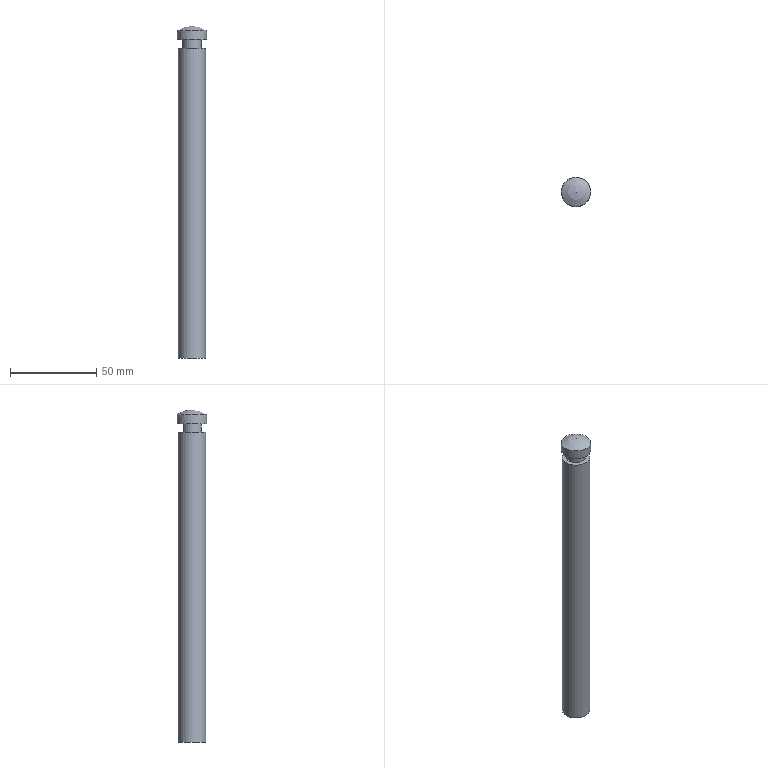Component | NX | STUD_B_2 | 1 solid | 7 faces | box 17 x 17 x 192 mm | volume 37991 mm3 | plane 3 | cylinder 3 | sphere 1 | commonest cylinder face diameters 16 x1 11 x1 17 x1
STEP:
#1=CARTESIAN_POINT('',(0.,0.,0.));
#2=DIRECTION('',(0.,0.,1.));
#3=DIRECTION('',(1.,0.,0.));
#4=AXIS2_PLACEMENT_3D('',#1,#2,#3);
#5=CARTESIAN_POINT('',(194.,-0.,10.));
#6=VERTEX_POINT('',#5);
#7=CARTESIAN_POINT('',(186.,-0.,10.));
#8=DIRECTION('',(0.,0.,1.));
#9=DIRECTION('',(1.,0.,0.));
#10=AXIS2_PLACEMENT_3D('',#7,#8,#9);
#11=CIRCLE('',#10,8.);
#12=CARTESIAN_POINT('',(186.,-0.,10.));
#13=DIRECTION('',(0.,0.,1.));
#14=DIRECTION('',(1.,0.,0.));
#15=AXIS2_PLACEMENT_3D('',#12,#13,#14);
#16=PLANE('',#15);
#17=CARTESIAN_POINT('',(0.,0.));
#18=DIRECTION('',(1.,0.));
#19=AXIS2_PLACEMENT_2D('',#17,#18);
#20=CIRCLE('',#19,8.);
#21=(GEOMETRIC_REPRESENTATION_CONTEXT(2)PARAMETRIC_REPRESENTATION_CONTEXT()REPRESENTATION_CONTEXT('',''));
#22=DEFINITIONAL_REPRESENTATION('',(#20),#21);
#23=PCURVE('',#16,#22);
#24=CARTESIAN_POINT('',(186.,-0.,202.));
#25=DIRECTION('',(0.,0.,1.));
#26=DIRECTION('',(1.,0.,0.));
#27=AXIS2_PLACEMENT_3D('',#24,#25,#26);
#28=CYLINDRICAL_SURFACE('',#27,8.);
#29=CARTESIAN_POINT('',(0.,-192.));
#30=DIRECTION('',(1.,0.));
#31=VECTOR('',#30,1.);
#32=LINE('',#29,#31);
#33=(GEOMETRIC_REPRESENTATION_CONTEXT(2)PARAMETRIC_REPRESENTATION_CONTEXT()REPRESENTATION_CONTEXT('',''));
#34=DEFINITIONAL_REPRESENTATION('',(#32),#33);
#35=PCURVE('',#28,#34);
#36=SURFACE_CURVE('',#11,(#23,#35),.PCURVE_S1.);
#37=EDGE_CURVE('',#6,#6,#36,.T.);
#38=ORIENTED_EDGE('',*,*,#37,.F.);
#39=EDGE_LOOP('',(#38));
#40=FACE_BOUND('',#39,.T.);
#41=ADVANCED_FACE('',(#40),#16,.F.);
#42=ORIENTED_EDGE('',*,*,#37,.T.);
#43=CARTESIAN_POINT('',(194.,-0.,189.));
#44=VERTEX_POINT('',#43);
#45=CARTESIAN_POINT('',(194.,-0.,10.));
#46=CARTESIAN_POINT('',(194.,-0.,189.));
#47=B_SPLINE_CURVE_WITH_KNOTS('',1,(#45,#46),.UNSPECIFIED.,.F.,.F.,(2,2),(-192.,-13.),.PIECEWISE_BEZIER_KNOTS.);
#48=CARTESIAN_POINT('',(6.283,0.));
#49=DIRECTION('',(0.,1.));
#50=VECTOR('',#49,1.);
#51=LINE('',#48,#50);
#52=(GEOMETRIC_REPRESENTATION_CONTEXT(2)PARAMETRIC_REPRESENTATION_CONTEXT()REPRESENTATION_CONTEXT('',''));
#53=DEFINITIONAL_REPRESENTATION('',(#51),#52);
#54=PCURVE('',#28,#53);
#55=CARTESIAN_POINT('',(0.,0.));
#56=DIRECTION('',(0.,1.));
#57=VECTOR('',#56,1.);
#58=LINE('',#55,#57);
#59=(GEOMETRIC_REPRESENTATION_CONTEXT(2)PARAMETRIC_REPRESENTATION_CONTEXT()REPRESENTATION_CONTEXT('',''));
#60=DEFINITIONAL_REPRESENTATION('',(#58),#59);
#61=PCURVE('',#28,#60);
#62=SEAM_CURVE('',#47,(#54,#61),.PCURVE_S1.);
#63=EDGE_CURVE('',#6,#44,#62,.T.);
#64=ORIENTED_EDGE('',*,*,#63,.T.);
#65=CARTESIAN_POINT('',(186.,-0.,189.));
#66=DIRECTION('',(0.,0.,1.));
#67=DIRECTION('',(1.,0.,0.));
#68=AXIS2_PLACEMENT_3D('',#65,#66,#67);
#69=CIRCLE('',#68,8.);
#70=CARTESIAN_POINT('',(0.,-13.));
#71=DIRECTION('',(1.,0.));
#72=VECTOR('',#71,1.);
#73=LINE('',#70,#72);
#74=(GEOMETRIC_REPRESENTATION_CONTEXT(2)PARAMETRIC_REPRESENTATION_CONTEXT()REPRESENTATION_CONTEXT('',''));
#75=DEFINITIONAL_REPRESENTATION('',(#73),#74);
#76=PCURVE('',#28,#75);
#77=CARTESIAN_POINT('',(186.,-5.5,189.));
#78=DIRECTION('',(0.,0.,1.));
#79=DIRECTION('',(1.,0.,0.));
#80=AXIS2_PLACEMENT_3D('',#77,#78,#79);
#81=PLANE('',#80);
#82=CARTESIAN_POINT('',(0.,5.5));
#83=DIRECTION('',(1.,0.));
#84=AXIS2_PLACEMENT_2D('',#82,#83);
#85=CIRCLE('',#84,8.);
#86=(GEOMETRIC_REPRESENTATION_CONTEXT(2)PARAMETRIC_REPRESENTATION_CONTEXT()REPRESENTATION_CONTEXT('',''));
#87=DEFINITIONAL_REPRESENTATION('',(#85),#86);
#88=PCURVE('',#81,#87);
#89=SURFACE_CURVE('',#69,(#76,#88),.PCURVE_S1.);
#90=EDGE_CURVE('',#44,#44,#89,.T.);
#91=ORIENTED_EDGE('',*,*,#90,.F.);
#92=ORIENTED_EDGE('',*,*,#63,.F.);
#93=EDGE_LOOP('',(#42,#64,#91,#92));
#94=FACE_BOUND('',#93,.T.);
#95=ADVANCED_FACE('',(#94),#28,.T.);
#96=ORIENTED_EDGE('',*,*,#90,.T.);
#97=EDGE_LOOP('',(#96));
#98=FACE_BOUND('',#97,.T.);
#99=CARTESIAN_POINT('',(191.5,-0.,189.));
#100=VERTEX_POINT('',#99);
#101=CARTESIAN_POINT('',(186.,-0.,189.));
#102=DIRECTION('',(0.,0.,1.));
#103=DIRECTION('',(1.,0.,0.));
#104=AXIS2_PLACEMENT_3D('',#101,#102,#103);
#105=CIRCLE('',#104,5.5);
#106=CARTESIAN_POINT('',(0.,5.5));
#107=DIRECTION('',(1.,0.));
#108=AXIS2_PLACEMENT_2D('',#106,#107);
#109=CIRCLE('',#108,5.5);
#110=(GEOMETRIC_REPRESENTATION_CONTEXT(2)PARAMETRIC_REPRESENTATION_CONTEXT()REPRESENTATION_CONTEXT('',''));
#111=DEFINITIONAL_REPRESENTATION('',(#109),#110);
#112=PCURVE('',#81,#111);
#113=CARTESIAN_POINT('',(186.,-0.,202.));
#114=DIRECTION('',(0.,0.,1.));
#115=DIRECTION('',(1.,0.,0.));
#116=AXIS2_PLACEMENT_3D('',#113,#114,#115);
#117=CYLINDRICAL_SURFACE('',#116,5.5);
#118=CARTESIAN_POINT('',(0.,-13.));
#119=DIRECTION('',(1.,0.));
#120=VECTOR('',#119,1.);
#121=LINE('',#118,#120);
#122=(GEOMETRIC_REPRESENTATION_CONTEXT(2)PARAMETRIC_REPRESENTATION_CONTEXT()REPRESENTATION_CONTEXT('',''));
#123=DEFINITIONAL_REPRESENTATION('',(#121),#122);
#124=PCURVE('',#117,#123);
#125=SURFACE_CURVE('',#105,(#112,#124),.PCURVE_S1.);
#126=EDGE_CURVE('',#100,#100,#125,.T.);
#127=ORIENTED_EDGE('',*,*,#126,.F.);
#128=EDGE_LOOP('',(#127));
#129=FACE_BOUND('',#128,.T.);
#130=ADVANCED_FACE('',(#98,#129),#81,.T.);
#131=ORIENTED_EDGE('',*,*,#126,.T.);
#132=CARTESIAN_POINT('',(191.5,-0.,194.));
#133=VERTEX_POINT('',#132);
#134=CARTESIAN_POINT('',(191.5,-0.,189.));
#135=CARTESIAN_POINT('',(191.5,-0.,194.));
#136=B_SPLINE_CURVE_WITH_KNOTS('',1,(#134,#135),.UNSPECIFIED.,.F.,.F.,(2,2),(-13.,-8.),.PIECEWISE_BEZIER_KNOTS.);
#137=CARTESIAN_POINT('',(6.283,0.));
#138=DIRECTION('',(0.,1.));
#139=VECTOR('',#138,1.);
#140=LINE('',#137,#139);
#141=(GEOMETRIC_REPRESENTATION_CONTEXT(2)PARAMETRIC_REPRESENTATION_CONTEXT()REPRESENTATION_CONTEXT('',''));
#142=DEFINITIONAL_REPRESENTATION('',(#140),#141);
#143=PCURVE('',#117,#142);
#144=CARTESIAN_POINT('',(0.,0.));
#145=DIRECTION('',(0.,1.));
#146=VECTOR('',#145,1.);
#147=LINE('',#144,#146);
#148=(GEOMETRIC_REPRESENTATION_CONTEXT(2)PARAMETRIC_REPRESENTATION_CONTEXT()REPRESENTATION_CONTEXT('',''));
#149=DEFINITIONAL_REPRESENTATION('',(#147),#148);
#150=PCURVE('',#117,#149);
#151=SEAM_CURVE('',#136,(#143,#150),.PCURVE_S1.);
#152=EDGE_CURVE('',#100,#133,#151,.T.);
#153=ORIENTED_EDGE('',*,*,#152,.T.);
#154=CARTESIAN_POINT('',(186.,-0.,194.));
#155=DIRECTION('',(0.,0.,1.));
#156=DIRECTION('',(1.,0.,0.));
#157=AXIS2_PLACEMENT_3D('',#154,#155,#156);
#158=CIRCLE('',#157,5.5);
#159=CARTESIAN_POINT('',(0.,-8.));
#160=DIRECTION('',(1.,0.));
#161=VECTOR('',#160,1.);
#162=LINE('',#159,#161);
#163=(GEOMETRIC_REPRESENTATION_CONTEXT(2)PARAMETRIC_REPRESENTATION_CONTEXT()REPRESENTATION_CONTEXT('',''));
#164=DEFINITIONAL_REPRESENTATION('',(#162),#163);
#165=PCURVE('',#117,#164);
#166=CARTESIAN_POINT('',(186.,-8.5,194.));
#167=DIRECTION('',(0.,0.,-1.));
#168=DIRECTION('',(-1.,0.,0.));
#169=AXIS2_PLACEMENT_3D('',#166,#167,#168);
#170=PLANE('',#169);
#171=CARTESIAN_POINT('',(-5.5,8.5));
#172=CARTESIAN_POINT('',(-5.5,18.026));
#173=CARTESIAN_POINT('',(2.75,13.263));
#174=CARTESIAN_POINT('',(11.,8.5));
#175=CARTESIAN_POINT('',(2.75,3.737));
#176=CARTESIAN_POINT('',(-5.5,-1.026));
#177=CARTESIAN_POINT('',(-5.5,8.5));
#178=(BOUNDED_CURVE()B_SPLINE_CURVE(2,(#171,#172,#173,#174,#175,#176,#177),.UNSPECIFIED.,.T.,.F.)B_SPLINE_CURVE_WITH_KNOTS((1,2,2,2,2,1),(-2.094,0.,2.094,4.189,6.283,8.378),.UNSPECIFIED.)CURVE()GEOMETRIC_REPRESENTATION_ITEM()RATIONAL_B_SPLINE_CURVE((1.,0.5,1.,0.5,1.,0.5,1.))REPRESENTATION_ITEM(''));
#179=(GEOMETRIC_REPRESENTATION_CONTEXT(2)PARAMETRIC_REPRESENTATION_CONTEXT()REPRESENTATION_CONTEXT('',''));
#180=DEFINITIONAL_REPRESENTATION('',(#178),#179);
#181=PCURVE('',#170,#180);
#182=SURFACE_CURVE('',#158,(#165,#181),.PCURVE_S1.);
#183=EDGE_CURVE('',#133,#133,#182,.T.);
#184=ORIENTED_EDGE('',*,*,#183,.F.);
#185=ORIENTED_EDGE('',*,*,#152,.F.);
#186=EDGE_LOOP('',(#131,#153,#184,#185));
#187=FACE_BOUND('',#186,.T.);
#188=ADVANCED_FACE('',(#187),#117,.T.);
#189=ORIENTED_EDGE('',*,*,#183,.T.);
#190=EDGE_LOOP('',(#189));
#191=FACE_BOUND('',#190,.T.);
#192=CARTESIAN_POINT('',(194.5,-0.,194.));
#193=VERTEX_POINT('',#192);
#194=CARTESIAN_POINT('',(186.,-0.,194.));
#195=DIRECTION('',(0.,0.,1.));
#196=DIRECTION('',(1.,0.,0.));
#197=AXIS2_PLACEMENT_3D('',#194,#195,#196);
#198=CIRCLE('',#197,8.5);
#199=CARTESIAN_POINT('',(-8.5,8.5));
#200=CARTESIAN_POINT('',(-8.5,23.222));
#201=CARTESIAN_POINT('',(4.25,15.861));
#202=CARTESIAN_POINT('',(17.,8.5));
#203=CARTESIAN_POINT('',(4.25,1.139));
#204=CARTESIAN_POINT('',(-8.5,-6.222));
#205=CARTESIAN_POINT('',(-8.5,8.5));
#206=(BOUNDED_CURVE()B_SPLINE_CURVE(2,(#199,#200,#201,#202,#203,#204,#205),.UNSPECIFIED.,.T.,.F.)B_SPLINE_CURVE_WITH_KNOTS((1,2,2,2,2,1),(-2.094,0.,2.094,4.189,6.283,8.378),.UNSPECIFIED.)CURVE()GEOMETRIC_REPRESENTATION_ITEM()RATIONAL_B_SPLINE_CURVE((1.,0.5,1.,0.5,1.,0.5,1.))REPRESENTATION_ITEM(''));
#207=(GEOMETRIC_REPRESENTATION_CONTEXT(2)PARAMETRIC_REPRESENTATION_CONTEXT()REPRESENTATION_CONTEXT('',''));
#208=DEFINITIONAL_REPRESENTATION('',(#206),#207);
#209=PCURVE('',#170,#208);
#210=CARTESIAN_POINT('',(186.,-0.,202.));
#211=DIRECTION('',(0.,0.,1.));
#212=DIRECTION('',(1.,0.,0.));
#213=AXIS2_PLACEMENT_3D('',#210,#211,#212);
#214=CYLINDRICAL_SURFACE('',#213,8.5);
#215=CARTESIAN_POINT('',(0.,-8.));
#216=DIRECTION('',(1.,0.));
#217=VECTOR('',#216,1.);
#218=LINE('',#215,#217);
#219=(GEOMETRIC_REPRESENTATION_CONTEXT(2)PARAMETRIC_REPRESENTATION_CONTEXT()REPRESENTATION_CONTEXT('',''));
#220=DEFINITIONAL_REPRESENTATION('',(#218),#219);
#221=PCURVE('',#214,#220);
#222=SURFACE_CURVE('',#198,(#209,#221),.PCURVE_S1.);
#223=EDGE_CURVE('',#193,#193,#222,.T.);
#224=ORIENTED_EDGE('',*,*,#223,.F.);
#225=EDGE_LOOP('',(#224));
#226=FACE_BOUND('',#225,.T.);
#227=ADVANCED_FACE('',(#191,#226),#170,.T.);
#228=ORIENTED_EDGE('',*,*,#223,.T.);
#229=CARTESIAN_POINT('',(194.5,-0.,199.359));
#230=VERTEX_POINT('',#229);
#231=CARTESIAN_POINT('',(194.5,-0.,194.));
#232=CARTESIAN_POINT('',(194.5,-0.,199.359));
#233=B_SPLINE_CURVE_WITH_KNOTS('',1,(#231,#232),.UNSPECIFIED.,.F.,.F.,(2,2),(-8.,-2.641),.PIECEWISE_BEZIER_KNOTS.);
#234=CARTESIAN_POINT('',(6.283,0.));
#235=DIRECTION('',(0.,1.));
#236=VECTOR('',#235,1.);
#237=LINE('',#234,#236);
#238=(GEOMETRIC_REPRESENTATION_CONTEXT(2)PARAMETRIC_REPRESENTATION_CONTEXT()REPRESENTATION_CONTEXT('',''));
#239=DEFINITIONAL_REPRESENTATION('',(#237),#238);
#240=PCURVE('',#214,#239);
#241=CARTESIAN_POINT('',(0.,0.));
#242=DIRECTION('',(0.,1.));
#243=VECTOR('',#242,1.);
#244=LINE('',#241,#243);
#245=(GEOMETRIC_REPRESENTATION_CONTEXT(2)PARAMETRIC_REPRESENTATION_CONTEXT()REPRESENTATION_CONTEXT('',''));
#246=DEFINITIONAL_REPRESENTATION('',(#244),#245);
#247=PCURVE('',#214,#246);
#248=SEAM_CURVE('',#233,(#240,#247),.PCURVE_S1.);
#249=EDGE_CURVE('',#193,#230,#248,.T.);
#250=ORIENTED_EDGE('',*,*,#249,.T.);
#251=CARTESIAN_POINT('',(186.,8.5,199.359));
#252=VERTEX_POINT('',#251);
#253=CARTESIAN_POINT('',(186.,-0.,199.359));
#254=DIRECTION('',(0.,0.,1.));
#255=DIRECTION('',(1.,0.,0.));
#256=AXIS2_PLACEMENT_3D('',#253,#254,#255);
#257=CIRCLE('',#256,8.5);
#258=CARTESIAN_POINT('',(0.,-2.641));
#259=DIRECTION('',(1.,0.));
#260=VECTOR('',#259,1.);
#261=LINE('',#258,#260);
#262=(GEOMETRIC_REPRESENTATION_CONTEXT(2)PARAMETRIC_REPRESENTATION_CONTEXT()REPRESENTATION_CONTEXT('',''));
#263=DEFINITIONAL_REPRESENTATION('',(#261),#262);
#264=PCURVE('',#214,#263);
#265=CARTESIAN_POINT('',(186.,-0.,187.));
#266=DIRECTION('',(0.,0.,1.));
#267=DIRECTION('',(0.,1.,-0.));
#268=AXIS2_PLACEMENT_3D('',#265,#266,#267);
#269=SPHERICAL_SURFACE('',#268,15.);
#270=CARTESIAN_POINT('',(-1.571,0.9683));
#271=CARTESIAN_POINT('',(-1.476,0.9683));
#272=CARTESIAN_POINT('',(-1.285,0.9683));
#273=CARTESIAN_POINT('',(-0.9996,0.9683));
#274=CARTESIAN_POINT('',(-0.714,0.9683));
#275=CARTESIAN_POINT('',(-0.4284,0.9683));
#276=CARTESIAN_POINT('',(-0.1428,0.9683));
#277=CARTESIAN_POINT('',(0.1428,0.9683));
#278=CARTESIAN_POINT('',(0.4284,0.9683));
#279=CARTESIAN_POINT('',(0.714,0.9683));
#280=CARTESIAN_POINT('',(0.9996,0.9683));
#281=CARTESIAN_POINT('',(1.285,0.9683));
#282=CARTESIAN_POINT('',(1.571,0.9683));
#283=CARTESIAN_POINT('',(1.856,0.9683));
#284=CARTESIAN_POINT('',(2.142,0.9683));
#285=CARTESIAN_POINT('',(2.428,0.9683));
#286=CARTESIAN_POINT('',(2.713,0.9683));
#287=CARTESIAN_POINT('',(2.999,0.9683));
#288=CARTESIAN_POINT('',(3.284,0.9683));
#289=CARTESIAN_POINT('',(3.57,0.9683));
#290=CARTESIAN_POINT('',(3.856,0.9683));
#291=CARTESIAN_POINT('',(4.141,0.9683));
#292=CARTESIAN_POINT('',(4.427,0.9683));
#293=CARTESIAN_POINT('',(4.617,0.9683));
#294=CARTESIAN_POINT('',(4.712,0.9683));
#295=B_SPLINE_CURVE_WITH_KNOTS('',3,(#270,#271,#272,#273,#274,#275,#276,#277,#278,#279,#280,#281,#282,#283,#284,#285,#286,#287,#288,#289,#290,#291,#292,#293,#294),.UNSPECIFIED.,.F.,.F.,(4,1,1,1,1,1,1,1,1,1,1,1,1,1,1,1,1,1,1,1,1,1,4),(0.,0.2856,0.5712,0.8568,1.142,1.428,1.714,1.999,2.285,2.57,2.856,3.142,3.427,3.713,3.998,4.284,4.57,4.855,5.141,5.426,5.712,5.998,6.283),.QUASI_UNIFORM_KNOTS.);
#296=(GEOMETRIC_REPRESENTATION_CONTEXT(2)PARAMETRIC_REPRESENTATION_CONTEXT()REPRESENTATION_CONTEXT('',''));
#297=DEFINITIONAL_REPRESENTATION('',(#295),#296);
#298=PCURVE('',#269,#297);
#299=SURFACE_CURVE('',#257,(#264,#298),.PCURVE_S1.);
#300=EDGE_CURVE('',#252,#230,#299,.T.);
#301=ORIENTED_EDGE('',*,*,#300,.F.);
#302=CARTESIAN_POINT('',(186.,-0.,199.359));
#303=DIRECTION('',(0.,0.,1.));
#304=DIRECTION('',(1.,0.,0.));
#305=AXIS2_PLACEMENT_3D('',#302,#303,#304);
#306=CIRCLE('',#305,8.5);
#307=CARTESIAN_POINT('',(0.,-2.641));
#308=DIRECTION('',(1.,0.));
#309=VECTOR('',#308,1.);
#310=LINE('',#307,#309);
#311=(GEOMETRIC_REPRESENTATION_CONTEXT(2)PARAMETRIC_REPRESENTATION_CONTEXT()REPRESENTATION_CONTEXT('',''));
#312=DEFINITIONAL_REPRESENTATION('',(#310),#311);
#313=PCURVE('',#214,#312);
#314=CARTESIAN_POINT('',(4.712,0.9683));
#315=CARTESIAN_POINT('',(4.808,0.9683));
#316=CARTESIAN_POINT('',(4.998,0.9683));
#317=CARTESIAN_POINT('',(5.284,0.9683));
#318=CARTESIAN_POINT('',(5.569,0.9683));
#319=CARTESIAN_POINT('',(5.855,0.9683));
#320=CARTESIAN_POINT('',(6.14,0.9683));
#321=CARTESIAN_POINT('',(6.426,0.9683));
#322=CARTESIAN_POINT('',(6.712,0.9683));
#323=CARTESIAN_POINT('',(6.997,0.9683));
#324=CARTESIAN_POINT('',(7.283,0.9683));
#325=CARTESIAN_POINT('',(7.568,0.9683));
#326=CARTESIAN_POINT('',(7.854,0.9683));
#327=CARTESIAN_POINT('',(8.14,0.9683));
#328=CARTESIAN_POINT('',(8.425,0.9683));
#329=CARTESIAN_POINT('',(8.711,0.9683));
#330=CARTESIAN_POINT('',(8.996,0.9683));
#331=CARTESIAN_POINT('',(9.282,0.9683));
#332=CARTESIAN_POINT('',(9.568,0.9683));
#333=CARTESIAN_POINT('',(9.853,0.9683));
#334=CARTESIAN_POINT('',(10.139,0.9683));
#335=CARTESIAN_POINT('',(10.424,0.9683));
#336=CARTESIAN_POINT('',(10.71,0.9683));
#337=CARTESIAN_POINT('',(10.9,0.9683));
#338=CARTESIAN_POINT('',(10.996,0.9683));
#339=B_SPLINE_CURVE_WITH_KNOTS('',3,(#314,#315,#316,#317,#318,#319,#320,#321,#322,#323,#324,#325,#326,#327,#328,#329,#330,#331,#332,#333,#334,#335,#336,#337,#338),.UNSPECIFIED.,.F.,.F.,(4,1,1,1,1,1,1,1,1,1,1,1,1,1,1,1,1,1,1,1,1,1,4),(0.,0.2856,0.5712,0.8568,1.142,1.428,1.714,1.999,2.285,2.57,2.856,3.142,3.427,3.713,3.998,4.284,4.57,4.855,5.141,5.426,5.712,5.998,6.283),.QUASI_UNIFORM_KNOTS.);
#340=(GEOMETRIC_REPRESENTATION_CONTEXT(2)PARAMETRIC_REPRESENTATION_CONTEXT()REPRESENTATION_CONTEXT('',''));
#341=DEFINITIONAL_REPRESENTATION('',(#339),#340);
#342=PCURVE('',#269,#341);
#343=SURFACE_CURVE('',#306,(#313,#342),.PCURVE_S1.);
#344=EDGE_CURVE('',#230,#252,#343,.T.);
#345=ORIENTED_EDGE('',*,*,#344,.F.);
#346=ORIENTED_EDGE('',*,*,#249,.F.);
#347=EDGE_LOOP('',(#228,#250,#301,#345,#346));
#348=FACE_BOUND('',#347,.T.);
#349=ADVANCED_FACE('',(#348),#214,.T.);
#350=ORIENTED_EDGE('',*,*,#344,.T.);
#351=CARTESIAN_POINT('',(186.,-0.,202.));
#352=VERTEX_POINT('',#351);
#353=CARTESIAN_POINT('',(186.,8.5,199.359));
#354=CARTESIAN_POINT('',(186.,7.011,200.383));
#355=CARTESIAN_POINT('',(186.,5.367,201.183));
#356=CARTESIAN_POINT('',(186.,3.615,201.728));
#357=CARTESIAN_POINT('',(186.,1.807,202.));
#358=CARTESIAN_POINT('',(186.,-0.,202.));
#359=B_SPLINE_CURVE_WITH_KNOTS('',5,(#353,#354,#355,#356,#357,#358),.UNSPECIFIED.,.F.,.F.,(6,6),(0.9683,1.571),.PIECEWISE_BEZIER_KNOTS.);
#360=CARTESIAN_POINT('',(6.283,0.));
#361=DIRECTION('',(0.,1.));
#362=VECTOR('',#361,1.);
#363=LINE('',#360,#362);
#364=(GEOMETRIC_REPRESENTATION_CONTEXT(2)PARAMETRIC_REPRESENTATION_CONTEXT()REPRESENTATION_CONTEXT('',''));
#365=DEFINITIONAL_REPRESENTATION('',(#363),#364);
#366=PCURVE('',#269,#365);
#367=CARTESIAN_POINT('',(0.,0.));
#368=DIRECTION('',(0.,1.));
#369=VECTOR('',#368,1.);
#370=LINE('',#367,#369);
#371=(GEOMETRIC_REPRESENTATION_CONTEXT(2)PARAMETRIC_REPRESENTATION_CONTEXT()REPRESENTATION_CONTEXT('',''));
#372=DEFINITIONAL_REPRESENTATION('',(#370),#371);
#373=PCURVE('',#269,#372);
#374=SEAM_CURVE('',#359,(#366,#373),.PCURVE_S1.);
#375=EDGE_CURVE('',#252,#352,#374,.T.);
#376=ORIENTED_EDGE('',*,*,#375,.T.);
#377=ORIENTED_EDGE('',*,*,#375,.F.);
#378=ORIENTED_EDGE('',*,*,#300,.T.);
#379=EDGE_LOOP('',(#350,#376,#377,#378));
#380=FACE_BOUND('',#379,.T.);
#381=ADVANCED_FACE('',(#380),#269,.T.);
#382=CLOSED_SHELL('',(#41,#95,#130,#188,#227,#349,#381));
#383=MANIFOLD_SOLID_BREP('',#382);
#384=(LENGTH_UNIT()NAMED_UNIT(*)SI_UNIT(.MILLI.,.METRE.));
#385=UNCERTAINTY_MEASURE_WITH_UNIT(LENGTH_MEASURE(0.00001),#384,'','');
#386=(NAMED_UNIT(*)PLANE_ANGLE_UNIT()SI_UNIT($,.RADIAN.));
#387=(NAMED_UNIT(*)SI_UNIT($,.STERADIAN.)SOLID_ANGLE_UNIT());
#388=(GEOMETRIC_REPRESENTATION_CONTEXT(3)GLOBAL_UNCERTAINTY_ASSIGNED_CONTEXT((#385))GLOBAL_UNIT_ASSIGNED_CONTEXT((#384,#386,#387))REPRESENTATION_CONTEXT('',''));
#389=ADVANCED_BREP_SHAPE_REPRESENTATION('',(#4,#383),#388);